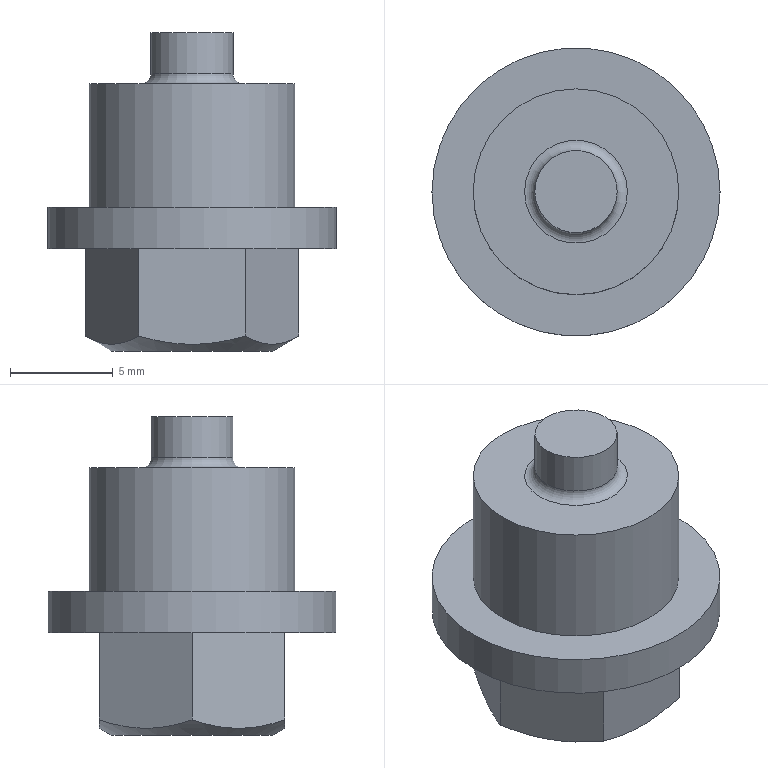Component | NX | ARM_TUBE_NUT | 1 solid | 16 faces | volume 1156 mm3 | plane 11 | cylinder 3 | torus 1 | cone 1 | commonest cylinder face diameters 4 x1 10 x1 14 x1